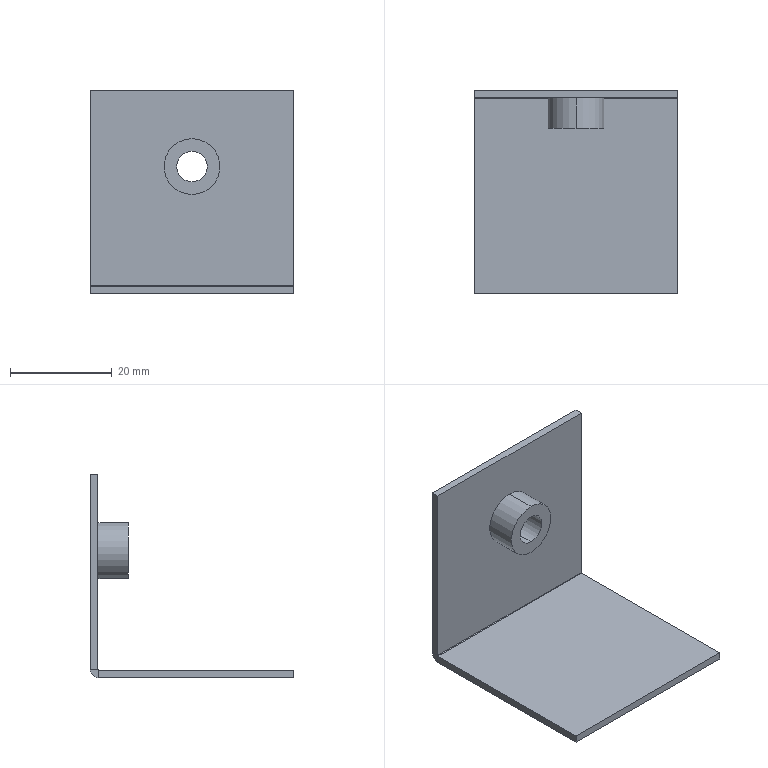Component | SolidWorks | CabinetWelding-1_MountingPlateBracket-1 | 1 solid | 22 faces | box 40 x 40 x 40 mm | volume 5013 mm3 | plane 14 | cylinder 8 | commonest cylinder face diameters 6 x2 11 x2 8 x2 3.2 x1 0.2 x1
STEP:
#1=CARTESIAN_POINT('',(11.302,-36.788,54.063));
#2=VERTEX_POINT('',#1);
#3=CARTESIAN_POINT('',(11.302,-36.788,54.299));
#4=VERTEX_POINT('',#3);
#5=CARTESIAN_POINT('',(11.302,-36.788,54.181));
#6=DIRECTION('',(0.,-1.,-0.));
#7=DIRECTION('',(0.,0.,1.));
#8=AXIS2_PLACEMENT_3D('',#5,#6,#7);
#9=CIRCLE('',#8,0.1181);
#10=EDGE_CURVE('',#2,#4,#9,.T.);
#11=ORIENTED_EDGE('',*,*,#10,.T.);
#12=CARTESIAN_POINT('',(11.302,-36.552,54.299));
#13=VERTEX_POINT('',#12);
#14=CARTESIAN_POINT('',(11.302,-36.788,54.299));
#15=DIRECTION('',(-0.,1.,0.));
#16=VECTOR('',#15,39.37);
#17=LINE('',#14,#16);
#18=EDGE_CURVE('',#4,#13,#17,.T.);
#19=ORIENTED_EDGE('',*,*,#18,.T.);
#20=CARTESIAN_POINT('',(11.302,-36.552,54.063));
#21=VERTEX_POINT('',#20);
#22=CARTESIAN_POINT('',(11.302,-36.552,54.181));
#23=DIRECTION('',(0.,-1.,-0.));
#24=DIRECTION('',(0.,0.,1.));
#25=AXIS2_PLACEMENT_3D('',#22,#23,#24);
#26=CIRCLE('',#25,0.1181);
#27=EDGE_CURVE('',#21,#13,#26,.T.);
#28=ORIENTED_EDGE('',*,*,#27,.F.);
#29=CARTESIAN_POINT('',(11.302,-36.788,54.063));
#30=DIRECTION('',(-0.,1.,0.));
#31=VECTOR('',#30,39.37);
#32=LINE('',#29,#31);
#33=EDGE_CURVE('',#2,#21,#32,.T.);
#34=ORIENTED_EDGE('',*,*,#33,.F.);
#35=EDGE_LOOP('',(#11,#19,#28,#34));
#36=FACE_OUTER_BOUND('',#35,.T.);
#37=CARTESIAN_POINT('',(11.302,-36.788,54.181));
#38=DIRECTION('',(-0.,1.,0.));
#39=DIRECTION('',(0.,0.,-1.));
#40=AXIS2_PLACEMENT_3D('',#37,#38,#39);
#41=CYLINDRICAL_SURFACE('',#40,0.1181);
#42=ADVANCED_FACE('',(#36),#41,.F.);
#43=CARTESIAN_POINT('',(11.302,-36.788,54.398));
#44=VERTEX_POINT('',#43);
#45=CARTESIAN_POINT('',(11.302,-36.788,53.965));
#46=VERTEX_POINT('',#45);
#47=CARTESIAN_POINT('',(11.302,-36.788,54.181));
#48=DIRECTION('',(0.,-1.,-0.));
#49=DIRECTION('',(0.,0.,1.));
#50=AXIS2_PLACEMENT_3D('',#47,#48,#49);
#51=CIRCLE('',#50,0.2165);
#52=EDGE_CURVE('',#44,#46,#51,.T.);
#53=ORIENTED_EDGE('',*,*,#52,.F.);
#54=CARTESIAN_POINT('',(11.302,-36.552,54.398));
#55=VERTEX_POINT('',#54);
#56=CARTESIAN_POINT('',(11.302,-36.788,54.398));
#57=DIRECTION('',(-0.,1.,0.));
#58=VECTOR('',#57,39.37);
#59=LINE('',#56,#58);
#60=EDGE_CURVE('',#44,#55,#59,.T.);
#61=ORIENTED_EDGE('',*,*,#60,.T.);
#62=CARTESIAN_POINT('',(11.302,-36.552,53.965));
#63=VERTEX_POINT('',#62);
#64=CARTESIAN_POINT('',(11.302,-36.552,54.181));
#65=DIRECTION('',(0.,-1.,-0.));
#66=DIRECTION('',(-1.,0.,0.));
#67=AXIS2_PLACEMENT_3D('',#64,#65,#66);
#68=CIRCLE('',#67,0.2165);
#69=EDGE_CURVE('',#55,#63,#68,.T.);
#70=ORIENTED_EDGE('',*,*,#69,.T.);
#71=CARTESIAN_POINT('',(11.302,-36.788,53.965));
#72=DIRECTION('',(-0.,1.,0.));
#73=VECTOR('',#72,39.37);
#74=LINE('',#71,#73);
#75=EDGE_CURVE('',#46,#63,#74,.T.);
#76=ORIENTED_EDGE('',*,*,#75,.F.);
#77=EDGE_LOOP('',(#53,#61,#70,#76));
#78=FACE_OUTER_BOUND('',#77,.T.);
#79=CARTESIAN_POINT('',(11.302,-36.788,54.181));
#80=DIRECTION('',(-0.,1.,0.));
#81=DIRECTION('',(-0.,0.,-1.));
#82=AXIS2_PLACEMENT_3D('',#79,#80,#81);
#83=CYLINDRICAL_SURFACE('',#82,0.2165);
#84=ADVANCED_FACE('',(#78),#83,.T.);
#85=CARTESIAN_POINT('',(11.46,-36.552,54.181));
#86=VERTEX_POINT('',#85);
#87=CARTESIAN_POINT('',(11.145,-36.552,54.181));
#88=VERTEX_POINT('',#87);
#89=CARTESIAN_POINT('',(11.302,-36.552,54.181));
#90=DIRECTION('',(-0.,1.,0.));
#91=DIRECTION('',(-1.,0.,0.));
#92=AXIS2_PLACEMENT_3D('',#89,#90,#91);
#93=CIRCLE('',#92,0.1575);
#94=EDGE_CURVE('',#86,#88,#93,.T.);
#95=ORIENTED_EDGE('',*,*,#94,.F.);
#96=CARTESIAN_POINT('',(11.46,-36.493,54.181));
#97=VERTEX_POINT('',#96);
#98=CARTESIAN_POINT('',(11.46,-36.887,54.181));
#99=DIRECTION('',(-0.,1.,0.));
#100=VECTOR('',#99,39.37);
#101=LINE('',#98,#100);
#102=EDGE_CURVE('',#86,#97,#101,.T.);
#103=ORIENTED_EDGE('',*,*,#102,.T.);
#104=CARTESIAN_POINT('',(11.145,-36.493,54.181));
#105=VERTEX_POINT('',#104);
#106=CARTESIAN_POINT('',(11.302,-36.493,54.181));
#107=DIRECTION('',(-0.,1.,0.));
#108=DIRECTION('',(-1.,0.,0.));
#109=AXIS2_PLACEMENT_3D('',#106,#107,#108);
#110=CIRCLE('',#109,0.1575);
#111=EDGE_CURVE('',#97,#105,#110,.T.);
#112=ORIENTED_EDGE('',*,*,#111,.T.);
#113=CARTESIAN_POINT('',(11.145,-36.887,54.181));
#114=DIRECTION('',(-0.,1.,0.));
#115=VECTOR('',#114,39.37);
#116=LINE('',#113,#115);
#117=EDGE_CURVE('',#88,#105,#116,.T.);
#118=ORIENTED_EDGE('',*,*,#117,.F.);
#119=EDGE_LOOP('',(#95,#103,#112,#118));
#120=FACE_OUTER_BOUND('',#119,.T.);
#121=CARTESIAN_POINT('',(11.302,-36.887,54.181));
#122=DIRECTION('',(-0.,1.,0.));
#123=DIRECTION('',(-1.,0.,0.));
#124=AXIS2_PLACEMENT_3D('',#121,#122,#123);
#125=CYLINDRICAL_SURFACE('',#124,0.1575);
#126=ADVANCED_FACE('',(#120),#125,.F.);
#127=CARTESIAN_POINT('',(12.09,-36.552,53.26));
#128=VERTEX_POINT('',#127);
#129=CARTESIAN_POINT('',(10.515,-36.552,53.26));
#130=VERTEX_POINT('',#129);
#131=CARTESIAN_POINT('',(12.09,-36.552,53.26));
#132=DIRECTION('',(-1.,-0.,0.));
#133=VECTOR('',#132,39.37);
#134=LINE('',#131,#133);
#135=EDGE_CURVE('',#128,#130,#134,.T.);
#136=ORIENTED_EDGE('',*,*,#135,.F.);
#137=CARTESIAN_POINT('',(12.09,-36.552,54.772));
#138=VERTEX_POINT('',#137);
#139=CARTESIAN_POINT('',(12.09,-36.552,54.772));
#140=DIRECTION('',(-0.,0.,-1.));
#141=VECTOR('',#140,39.37);
#142=LINE('',#139,#141);
#143=EDGE_CURVE('',#138,#128,#142,.T.);
#144=ORIENTED_EDGE('',*,*,#143,.F.);
#145=CARTESIAN_POINT('',(10.515,-36.552,54.772));
#146=VERTEX_POINT('',#145);
#147=CARTESIAN_POINT('',(12.09,-36.552,54.772));
#148=DIRECTION('',(1.,0.,-0.));
#149=VECTOR('',#148,39.37);
#150=LINE('',#147,#149);
#151=EDGE_CURVE('',#146,#138,#150,.T.);
#152=ORIENTED_EDGE('',*,*,#151,.F.);
#153=CARTESIAN_POINT('',(10.515,-36.552,54.772));
#154=DIRECTION('',(0.,-0.,1.));
#155=VECTOR('',#154,39.37);
#156=LINE('',#153,#155);
#157=EDGE_CURVE('',#130,#146,#156,.T.);
#158=ORIENTED_EDGE('',*,*,#157,.F.);
#159=EDGE_LOOP('',(#136,#144,#152,#158));
#160=FACE_OUTER_BOUND('',#159,.T.);
#161=CARTESIAN_POINT('',(11.302,-36.552,54.181));
#162=DIRECTION('',(0.,-1.,-0.));
#163=DIRECTION('',(-1.,0.,0.));
#164=AXIS2_PLACEMENT_3D('',#161,#162,#163);
#165=CIRCLE('',#164,0.2165);
#166=EDGE_CURVE('',#63,#55,#165,.T.);
#167=ORIENTED_EDGE('',*,*,#166,.F.);
#168=ORIENTED_EDGE('',*,*,#69,.F.);
#169=EDGE_LOOP('',(#167,#168));
#170=FACE_BOUND('',#169,.T.);
#171=CARTESIAN_POINT('',(11.33,-36.552,53.333));
#172=DIRECTION('',(-0.,1.,0.));
#173=DIRECTION('',(-1.,-0.,0.));
#174=AXIS2_PLACEMENT_3D('',#171,#172,#173);
#175=PLANE('',#174);
#176=ADVANCED_FACE('',(#160,#170),#175,.F.);
#177=ORIENTED_EDGE('',*,*,#143,.T.);
#178=CARTESIAN_POINT('',(12.09,-36.493,53.26));
#179=VERTEX_POINT('',#178);
#180=CARTESIAN_POINT('',(12.09,-36.552,53.26));
#181=DIRECTION('',(-0.,1.,0.));
#182=VECTOR('',#181,39.37);
#183=LINE('',#180,#182);
#184=EDGE_CURVE('',#128,#179,#183,.T.);
#185=ORIENTED_EDGE('',*,*,#184,.T.);
#186=CARTESIAN_POINT('',(12.09,-36.493,54.772));
#187=VERTEX_POINT('',#186);
#188=CARTESIAN_POINT('',(12.09,-36.493,54.772));
#189=DIRECTION('',(-0.,0.,-1.));
#190=VECTOR('',#189,39.37);
#191=LINE('',#188,#190);
#192=EDGE_CURVE('',#187,#179,#191,.T.);
#193=ORIENTED_EDGE('',*,*,#192,.F.);
#194=CARTESIAN_POINT('',(12.09,-36.552,54.772));
#195=DIRECTION('',(-0.,1.,0.));
#196=VECTOR('',#195,39.37);
#197=LINE('',#194,#196);
#198=EDGE_CURVE('',#138,#187,#197,.T.);
#199=ORIENTED_EDGE('',*,*,#198,.F.);
#200=EDGE_LOOP('',(#177,#185,#193,#199));
#201=FACE_OUTER_BOUND('',#200,.T.);
#202=CARTESIAN_POINT('',(12.09,-36.552,54.772));
#203=DIRECTION('',(1.,0.,-0.));
#204=DIRECTION('',(-0.,0.,-1.));
#205=AXIS2_PLACEMENT_3D('',#202,#203,#204);
#206=PLANE('',#205);
#207=ADVANCED_FACE('',(#201),#206,.T.);
#208=CARTESIAN_POINT('',(11.302,-36.493,54.181));
#209=DIRECTION('',(-0.,1.,0.));
#210=DIRECTION('',(-1.,0.,0.));
#211=AXIS2_PLACEMENT_3D('',#208,#209,#210);
#212=CIRCLE('',#211,0.1575);
#213=EDGE_CURVE('',#105,#97,#212,.T.);
#214=ORIENTED_EDGE('',*,*,#213,.F.);
#215=ORIENTED_EDGE('',*,*,#111,.F.);
#216=EDGE_LOOP('',(#214,#215));
#217=FACE_BOUND('',#216,.T.);
#218=ORIENTED_EDGE('',*,*,#192,.T.);
#219=CARTESIAN_POINT('',(10.515,-36.493,53.26));
#220=VERTEX_POINT('',#219);
#221=CARTESIAN_POINT('',(12.09,-36.493,53.26));
#222=DIRECTION('',(-1.,-0.,0.));
#223=VECTOR('',#222,39.37);
#224=LINE('',#221,#223);
#225=EDGE_CURVE('',#179,#220,#224,.T.);
#226=ORIENTED_EDGE('',*,*,#225,.T.);
#227=CARTESIAN_POINT('',(10.515,-36.493,54.772));
#228=VERTEX_POINT('',#227);
#229=CARTESIAN_POINT('',(10.515,-36.493,54.772));
#230=DIRECTION('',(0.,-0.,1.));
#231=VECTOR('',#230,39.37);
#232=LINE('',#229,#231);
#233=EDGE_CURVE('',#220,#228,#232,.T.);
#234=ORIENTED_EDGE('',*,*,#233,.T.);
#235=CARTESIAN_POINT('',(12.09,-36.493,54.772));
#236=DIRECTION('',(1.,0.,-0.));
#237=VECTOR('',#236,39.37);
#238=LINE('',#235,#237);
#239=EDGE_CURVE('',#228,#187,#238,.T.);
#240=ORIENTED_EDGE('',*,*,#239,.T.);
#241=EDGE_LOOP('',(#218,#226,#234,#240));
#242=FACE_OUTER_BOUND('',#241,.T.);
#243=CARTESIAN_POINT('',(11.33,-36.493,53.333));
#244=DIRECTION('',(-0.,1.,0.));
#245=DIRECTION('',(-1.,-0.,0.));
#246=AXIS2_PLACEMENT_3D('',#243,#244,#245);
#247=PLANE('',#246);
#248=ADVANCED_FACE('',(#217,#242),#247,.T.);
#249=ORIENTED_EDGE('',*,*,#239,.F.);
#250=CARTESIAN_POINT('',(10.515,-36.552,54.772));
#251=DIRECTION('',(-0.,1.,0.));
#252=VECTOR('',#251,39.37);
#253=LINE('',#250,#252);
#254=EDGE_CURVE('',#146,#228,#253,.T.);
#255=ORIENTED_EDGE('',*,*,#254,.F.);
#256=ORIENTED_EDGE('',*,*,#151,.T.);
#257=ORIENTED_EDGE('',*,*,#198,.T.);
#258=EDGE_LOOP('',(#249,#255,#256,#257));
#259=FACE_OUTER_BOUND('',#258,.T.);
#260=CARTESIAN_POINT('',(12.09,-36.552,54.772));
#261=DIRECTION('',(0.,-0.,1.));
#262=DIRECTION('',(-0.,1.,0.));
#263=AXIS2_PLACEMENT_3D('',#260,#261,#262);
#264=PLANE('',#263);
#265=ADVANCED_FACE('',(#259),#264,.T.);
#266=CARTESIAN_POINT('',(10.515,-36.552,53.26));
#267=DIRECTION('',(-0.,1.,0.));
#268=VECTOR('',#267,39.37);
#269=LINE('',#266,#268);
#270=EDGE_CURVE('',#130,#220,#269,.T.);
#271=ORIENTED_EDGE('',*,*,#270,.F.);
#272=ORIENTED_EDGE('',*,*,#157,.T.);
#273=ORIENTED_EDGE('',*,*,#254,.T.);
#274=ORIENTED_EDGE('',*,*,#233,.F.);
#275=EDGE_LOOP('',(#271,#272,#273,#274));
#276=FACE_OUTER_BOUND('',#275,.T.);
#277=CARTESIAN_POINT('',(10.515,-36.552,54.772));
#278=DIRECTION('',(-1.,-0.,0.));
#279=DIRECTION('',(0.,-0.,1.));
#280=AXIS2_PLACEMENT_3D('',#277,#278,#279);
#281=PLANE('',#280);
#282=ADVANCED_FACE('',(#276),#281,.T.);
#283=CARTESIAN_POINT('',(10.515,-36.556,53.256));
#284=VERTEX_POINT('',#283);
#285=CARTESIAN_POINT('',(10.515,-36.556,53.197));
#286=VERTEX_POINT('',#285);
#287=CARTESIAN_POINT('',(10.515,-36.556,53.197));
#288=DIRECTION('',(-0.,0.,-1.));
#289=VECTOR('',#288,39.37);
#290=LINE('',#287,#289);
#291=EDGE_CURVE('',#284,#286,#290,.T.);
#292=ORIENTED_EDGE('',*,*,#291,.F.);
#293=CARTESIAN_POINT('',(10.515,-36.556,53.26));
#294=DIRECTION('',(-1.,-0.,0.));
#295=DIRECTION('',(0.,1.,0.));
#296=AXIS2_PLACEMENT_3D('',#293,#294,#295);
#297=CIRCLE('',#296,0.003937);
#298=EDGE_CURVE('',#130,#284,#297,.T.);
#299=ORIENTED_EDGE('',*,*,#298,.F.);
#300=ORIENTED_EDGE('',*,*,#270,.T.);
#301=CARTESIAN_POINT('',(10.515,-36.556,53.26));
#302=DIRECTION('',(-1.,-0.,0.));
#303=DIRECTION('',(0.,1.,0.));
#304=AXIS2_PLACEMENT_3D('',#301,#302,#303);
#305=CIRCLE('',#304,0.06299);
#306=EDGE_CURVE('',#220,#286,#305,.T.);
#307=ORIENTED_EDGE('',*,*,#306,.T.);
#308=EDGE_LOOP('',(#292,#299,#300,#307));
#309=FACE_OUTER_BOUND('',#308,.T.);
#310=CARTESIAN_POINT('',(10.515,-36.556,53.26));
#311=DIRECTION('',(-1.,-0.,0.));
#312=DIRECTION('',(0.,-1.,-0.));
#313=AXIS2_PLACEMENT_3D('',#310,#311,#312);
#314=PLANE('',#313);
#315=ADVANCED_FACE('',(#309),#314,.T.);
#316=CARTESIAN_POINT('',(12.09,-36.556,53.256));
#317=VERTEX_POINT('',#316);
#318=CARTESIAN_POINT('',(12.09,-36.556,53.26));
#319=DIRECTION('',(1.,0.,-0.));
#320=DIRECTION('',(0.,1.,0.));
#321=AXIS2_PLACEMENT_3D('',#318,#319,#320);
#322=CIRCLE('',#321,0.003937);
#323=EDGE_CURVE('',#317,#128,#322,.T.);
#324=ORIENTED_EDGE('',*,*,#323,.F.);
#325=CARTESIAN_POINT('',(12.09,-36.556,53.197));
#326=VERTEX_POINT('',#325);
#327=CARTESIAN_POINT('',(12.09,-36.556,53.256));
#328=DIRECTION('',(-0.,0.,-1.));
#329=VECTOR('',#328,39.37);
#330=LINE('',#327,#329);
#331=EDGE_CURVE('',#317,#326,#330,.T.);
#332=ORIENTED_EDGE('',*,*,#331,.T.);
#333=CARTESIAN_POINT('',(12.09,-36.556,53.26));
#334=DIRECTION('',(1.,0.,-0.));
#335=DIRECTION('',(0.,1.,0.));
#336=AXIS2_PLACEMENT_3D('',#333,#334,#335);
#337=CIRCLE('',#336,0.06299);
#338=EDGE_CURVE('',#326,#179,#337,.T.);
#339=ORIENTED_EDGE('',*,*,#338,.T.);
#340=ORIENTED_EDGE('',*,*,#184,.F.);
#341=EDGE_LOOP('',(#324,#332,#339,#340));
#342=FACE_OUTER_BOUND('',#341,.T.);
#343=CARTESIAN_POINT('',(12.09,-36.556,53.26));
#344=DIRECTION('',(-1.,-0.,0.));
#345=DIRECTION('',(0.,-1.,-0.));
#346=AXIS2_PLACEMENT_3D('',#343,#344,#345);
#347=PLANE('',#346);
#348=ADVANCED_FACE('',(#342),#347,.F.);
#349=ORIENTED_EDGE('',*,*,#225,.F.);
#350=ORIENTED_EDGE('',*,*,#338,.F.);
#351=CARTESIAN_POINT('',(11.33,-36.556,53.197));
#352=DIRECTION('',(1.,0.,-0.));
#353=VECTOR('',#352,39.37);
#354=LINE('',#351,#353);
#355=EDGE_CURVE('',#286,#326,#354,.T.);
#356=ORIENTED_EDGE('',*,*,#355,.F.);
#357=ORIENTED_EDGE('',*,*,#306,.F.);
#358=EDGE_LOOP('',(#349,#350,#356,#357));
#359=FACE_OUTER_BOUND('',#358,.T.);
#360=CARTESIAN_POINT('',(12.09,-36.556,53.26));
#361=DIRECTION('',(1.,0.,-0.));
#362=DIRECTION('',(0.,0.,-1.));
#363=AXIS2_PLACEMENT_3D('',#360,#361,#362);
#364=CYLINDRICAL_SURFACE('',#363,0.06299);
#365=ADVANCED_FACE('',(#359),#364,.T.);
#366=ORIENTED_EDGE('',*,*,#135,.T.);
#367=ORIENTED_EDGE('',*,*,#298,.T.);
#368=CARTESIAN_POINT('',(10.515,-36.556,53.256));
#369=DIRECTION('',(1.,0.,-0.));
#370=VECTOR('',#369,39.37);
#371=LINE('',#368,#370);
#372=EDGE_CURVE('',#284,#317,#371,.T.);
#373=ORIENTED_EDGE('',*,*,#372,.T.);
#374=ORIENTED_EDGE('',*,*,#323,.T.);
#375=EDGE_LOOP('',(#366,#367,#373,#374));
#376=FACE_OUTER_BOUND('',#375,.T.);
#377=CARTESIAN_POINT('',(12.09,-36.556,53.26));
#378=DIRECTION('',(1.,0.,-0.));
#379=DIRECTION('',(0.,0.,-1.));
#380=AXIS2_PLACEMENT_3D('',#377,#378,#379);
#381=CYLINDRICAL_SURFACE('',#380,0.003937);
#382=ADVANCED_FACE('',(#376),#381,.F.);
#383=CARTESIAN_POINT('',(12.09,-38.068,53.197));
#384=VERTEX_POINT('',#383);
#385=CARTESIAN_POINT('',(12.09,-36.552,53.197));
#386=DIRECTION('',(-0.,1.,0.));
#387=VECTOR('',#386,39.37);
#388=LINE('',#385,#387);
#389=EDGE_CURVE('',#384,#326,#388,.T.);
#390=ORIENTED_EDGE('',*,*,#389,.T.);
#391=ORIENTED_EDGE('',*,*,#331,.F.);
#392=CARTESIAN_POINT('',(12.09,-38.068,53.256));
#393=VERTEX_POINT('',#392);
#394=CARTESIAN_POINT('',(12.09,-36.493,53.256));
#395=DIRECTION('',(-0.,1.,0.));
#396=VECTOR('',#395,39.37);
#397=LINE('',#394,#396);
#398=EDGE_CURVE('',#393,#317,#397,.T.);
#399=ORIENTED_EDGE('',*,*,#398,.F.);
#400=CARTESIAN_POINT('',(12.09,-38.068,53.197));
#401=DIRECTION('',(0.,-0.,1.));
#402=VECTOR('',#401,39.37);
#403=LINE('',#400,#402);
#404=EDGE_CURVE('',#384,#393,#403,.T.);
#405=ORIENTED_EDGE('',*,*,#404,.F.);
#406=EDGE_LOOP('',(#390,#391,#399,#405));
#407=FACE_OUTER_BOUND('',#406,.T.);
#408=CARTESIAN_POINT('',(12.09,-36.552,53.197));
#409=DIRECTION('',(1.,0.,-0.));
#410=DIRECTION('',(-0.,1.,0.));
#411=AXIS2_PLACEMENT_3D('',#408,#409,#410);
#412=PLANE('',#411);
#413=ADVANCED_FACE('',(#407),#412,.T.);
#414=CARTESIAN_POINT('',(10.515,-38.068,53.256));
#415=VERTEX_POINT('',#414);
#416=CARTESIAN_POINT('',(10.515,-36.493,53.256));
#417=DIRECTION('',(0.,-1.,-0.));
#418=VECTOR('',#417,39.37);
#419=LINE('',#416,#418);
#420=EDGE_CURVE('',#284,#415,#419,.T.);
#421=ORIENTED_EDGE('',*,*,#420,.F.);
#422=ORIENTED_EDGE('',*,*,#291,.T.);
#423=CARTESIAN_POINT('',(10.515,-38.068,53.197));
#424=VERTEX_POINT('',#423);
#425=CARTESIAN_POINT('',(10.515,-38.068,53.197));
#426=DIRECTION('',(0.,-1.,-0.));
#427=VECTOR('',#426,39.37);
#428=LINE('',#425,#427);
#429=EDGE_CURVE('',#286,#424,#428,.T.);
#430=ORIENTED_EDGE('',*,*,#429,.T.);
#431=CARTESIAN_POINT('',(10.515,-38.068,53.197));
#432=DIRECTION('',(0.,-0.,1.));
#433=VECTOR('',#432,39.37);
#434=LINE('',#431,#433);
#435=EDGE_CURVE('',#424,#415,#434,.T.);
#436=ORIENTED_EDGE('',*,*,#435,.T.);
#437=EDGE_LOOP('',(#421,#422,#430,#436));
#438=FACE_OUTER_BOUND('',#437,.T.);
#439=CARTESIAN_POINT('',(10.515,-38.068,53.197));
#440=DIRECTION('',(-1.,-0.,0.));
#441=DIRECTION('',(0.,-1.,-0.));
#442=AXIS2_PLACEMENT_3D('',#439,#440,#441);
#443=PLANE('',#442);
#444=ADVANCED_FACE('',(#438),#443,.T.);
#445=ORIENTED_EDGE('',*,*,#429,.F.);
#446=ORIENTED_EDGE('',*,*,#355,.T.);
#447=ORIENTED_EDGE('',*,*,#389,.F.);
#448=CARTESIAN_POINT('',(12.09,-38.068,53.197));
#449=DIRECTION('',(1.,0.,-0.));
#450=VECTOR('',#449,39.37);
#451=LINE('',#448,#450);
#452=EDGE_CURVE('',#424,#384,#451,.T.);
#453=ORIENTED_EDGE('',*,*,#452,.F.);
#454=EDGE_LOOP('',(#445,#446,#447,#453));
#455=FACE_OUTER_BOUND('',#454,.T.);
#456=CARTESIAN_POINT('',(11.33,-36.493,53.197));
#457=DIRECTION('',(-0.,0.,-1.));
#458=DIRECTION('',(0.,-1.,-0.));
#459=AXIS2_PLACEMENT_3D('',#456,#457,#458);
#460=PLANE('',#459);
#461=ADVANCED_FACE('',(#455),#460,.T.);
#462=ORIENTED_EDGE('',*,*,#372,.F.);
#463=ORIENTED_EDGE('',*,*,#420,.T.);
#464=CARTESIAN_POINT('',(11.33,-38.068,53.256));
#465=DIRECTION('',(1.,0.,-0.));
#466=VECTOR('',#465,39.37);
#467=LINE('',#464,#466);
#468=EDGE_CURVE('',#415,#393,#467,.T.);
#469=ORIENTED_EDGE('',*,*,#468,.T.);
#470=ORIENTED_EDGE('',*,*,#398,.T.);
#471=EDGE_LOOP('',(#462,#463,#469,#470));
#472=FACE_OUTER_BOUND('',#471,.T.);
#473=CARTESIAN_POINT('',(11.33,-36.493,53.256));
#474=DIRECTION('',(-0.,0.,-1.));
#475=DIRECTION('',(0.,-1.,-0.));
#476=AXIS2_PLACEMENT_3D('',#473,#474,#475);
#477=PLANE('',#476);
#478=ADVANCED_FACE('',(#472),#477,.F.);
#479=ORIENTED_EDGE('',*,*,#468,.F.);
#480=ORIENTED_EDGE('',*,*,#435,.F.);
#481=ORIENTED_EDGE('',*,*,#452,.T.);
#482=ORIENTED_EDGE('',*,*,#404,.T.);
#483=EDGE_LOOP('',(#479,#480,#481,#482));
#484=FACE_OUTER_BOUND('',#483,.T.);
#485=CARTESIAN_POINT('',(12.09,-38.068,53.197));
#486=DIRECTION('',(0.,-1.,-0.));
#487=DIRECTION('',(0.,-0.,1.));
#488=AXIS2_PLACEMENT_3D('',#485,#486,#487);
#489=PLANE('',#488);
#490=ADVANCED_FACE('',(#484),#489,.T.);
#491=ORIENTED_EDGE('',*,*,#102,.F.);
#492=CARTESIAN_POINT('',(11.302,-36.552,54.181));
#493=DIRECTION('',(-0.,1.,0.));
#494=DIRECTION('',(-1.,0.,0.));
#495=AXIS2_PLACEMENT_3D('',#492,#493,#494);
#496=CIRCLE('',#495,0.1575);
#497=EDGE_CURVE('',#88,#86,#496,.T.);
#498=ORIENTED_EDGE('',*,*,#497,.F.);
#499=ORIENTED_EDGE('',*,*,#117,.T.);
#500=ORIENTED_EDGE('',*,*,#213,.T.);
#501=EDGE_LOOP('',(#491,#498,#499,#500));
#502=FACE_OUTER_BOUND('',#501,.T.);
#503=CARTESIAN_POINT('',(11.302,-36.887,54.181));
#504=DIRECTION('',(-0.,1.,0.));
#505=DIRECTION('',(-1.,0.,0.));
#506=AXIS2_PLACEMENT_3D('',#503,#504,#505);
#507=CYLINDRICAL_SURFACE('',#506,0.1575);
#508=ADVANCED_FACE('',(#502),#507,.F.);
#509=ORIENTED_EDGE('',*,*,#27,.T.);
#510=CARTESIAN_POINT('',(11.302,-36.552,54.181));
#511=DIRECTION('',(0.,-1.,-0.));
#512=DIRECTION('',(0.,0.,1.));
#513=AXIS2_PLACEMENT_3D('',#510,#511,#512);
#514=CIRCLE('',#513,0.1181);
#515=EDGE_CURVE('',#13,#21,#514,.T.);
#516=ORIENTED_EDGE('',*,*,#515,.T.);
#517=EDGE_LOOP('',(#509,#516));
#518=FACE_BOUND('',#517,.T.);
#519=ORIENTED_EDGE('',*,*,#497,.T.);
#520=ORIENTED_EDGE('',*,*,#94,.T.);
#521=EDGE_LOOP('',(#519,#520));
#522=FACE_OUTER_BOUND('',#521,.T.);
#523=CARTESIAN_POINT('',(11.302,-36.552,54.181));
#524=DIRECTION('',(0.,-1.,-0.));
#525=DIRECTION('',(0.,-0.,1.));
#526=AXIS2_PLACEMENT_3D('',#523,#524,#525);
#527=PLANE('',#526);
#528=ADVANCED_FACE('',(#518,#522),#527,.F.);
#529=CARTESIAN_POINT('',(11.302,-36.788,54.181));
#530=DIRECTION('',(0.,-1.,-0.));
#531=DIRECTION('',(0.,0.,1.));
#532=AXIS2_PLACEMENT_3D('',#529,#530,#531);
#533=CIRCLE('',#532,0.2165);
#534=EDGE_CURVE('',#46,#44,#533,.T.);
#535=ORIENTED_EDGE('',*,*,#534,.T.);
#536=ORIENTED_EDGE('',*,*,#52,.T.);
#537=EDGE_LOOP('',(#535,#536));
#538=FACE_OUTER_BOUND('',#537,.T.);
#539=ORIENTED_EDGE('',*,*,#10,.F.);
#540=CARTESIAN_POINT('',(11.302,-36.788,54.181));
#541=DIRECTION('',(0.,-1.,-0.));
#542=DIRECTION('',(0.,0.,1.));
#543=AXIS2_PLACEMENT_3D('',#540,#541,#542);
#544=CIRCLE('',#543,0.1181);
#545=EDGE_CURVE('',#4,#2,#544,.T.);
#546=ORIENTED_EDGE('',*,*,#545,.F.);
#547=EDGE_LOOP('',(#539,#546));
#548=FACE_BOUND('',#547,.T.);
#549=CARTESIAN_POINT('',(11.302,-36.788,54.181));
#550=DIRECTION('',(0.,-1.,-0.));
#551=DIRECTION('',(0.,-0.,1.));
#552=AXIS2_PLACEMENT_3D('',#549,#550,#551);
#553=PLANE('',#552);
#554=ADVANCED_FACE('',(#538,#548),#553,.T.);
#555=ORIENTED_EDGE('',*,*,#60,.F.);
#556=ORIENTED_EDGE('',*,*,#534,.F.);
#557=ORIENTED_EDGE('',*,*,#75,.T.);
#558=ORIENTED_EDGE('',*,*,#166,.T.);
#559=EDGE_LOOP('',(#555,#556,#557,#558));
#560=FACE_OUTER_BOUND('',#559,.T.);
#561=CARTESIAN_POINT('',(11.302,-36.788,54.181));
#562=DIRECTION('',(-0.,1.,0.));
#563=DIRECTION('',(-0.,0.,-1.));
#564=AXIS2_PLACEMENT_3D('',#561,#562,#563);
#565=CYLINDRICAL_SURFACE('',#564,0.2165);
#566=ADVANCED_FACE('',(#560),#565,.T.);
#567=ORIENTED_EDGE('',*,*,#18,.F.);
#568=ORIENTED_EDGE('',*,*,#545,.T.);
#569=ORIENTED_EDGE('',*,*,#33,.T.);
#570=ORIENTED_EDGE('',*,*,#515,.F.);
#571=EDGE_LOOP('',(#567,#568,#569,#570));
#572=FACE_OUTER_BOUND('',#571,.T.);
#573=CARTESIAN_POINT('',(11.302,-36.788,54.181));
#574=DIRECTION('',(-0.,1.,0.));
#575=DIRECTION('',(0.,0.,-1.));
#576=AXIS2_PLACEMENT_3D('',#573,#574,#575);
#577=CYLINDRICAL_SURFACE('',#576,0.1181);
#578=ADVANCED_FACE('',(#572),#577,.F.);
#579=CLOSED_SHELL('',(#42,#84,#126,#176,#207,#248,#265,#282,#315,#348,#365,#382,#413,#444,#461,#478,#490,#508,#528,#554,#566,#578));
#580=MANIFOLD_SOLID_BREP('',#579);
#581=CARTESIAN_POINT('',(0.,0.,0.));
#582=DIRECTION('',(0.,0.,1.));
#583=DIRECTION('',(1.,0.,0.));
#584=AXIS2_PLACEMENT_3D('',#581,#582,#583);
#585=(LENGTH_UNIT()NAMED_UNIT(*)SI_UNIT($,.METRE.));
#586=LENGTH_MEASURE_WITH_UNIT(LENGTH_MEASURE(0.0254),#585);
#587=DIMENSIONAL_EXPONENTS(1.,0.,0.,0.,0.,0.,0.);
#588=(CONVERSION_BASED_UNIT('',#586)LENGTH_UNIT()NAMED_UNIT(#587));
#589=UNCERTAINTY_MEASURE_WITH_UNIT(LENGTH_MEASURE(0.00001),#588,'','');
#590=(NAMED_UNIT(*)PLANE_ANGLE_UNIT()SI_UNIT($,.RADIAN.));
#591=(NAMED_UNIT(*)SI_UNIT($,.STERADIAN.)SOLID_ANGLE_UNIT());
#592=(GEOMETRIC_REPRESENTATION_CONTEXT(3)GLOBAL_UNCERTAINTY_ASSIGNED_CONTEXT((#589))GLOBAL_UNIT_ASSIGNED_CONTEXT((#588,#590,#591))REPRESENTATION_CONTEXT('',''));
#593=ADVANCED_BREP_SHAPE_REPRESENTATION('',(#580,#584),#592);
#594=COLOUR_RGB('',0.7922,0.8196,0.9333);
#595=FILL_AREA_STYLE_COLOUR('',#594);
#596=FILL_AREA_STYLE('',(#595));
#597=SURFACE_STYLE_FILL_AREA(#596);
#598=SURFACE_SIDE_STYLE('',(#597));
#599=SURFACE_STYLE_USAGE(.BOTH.,#598);
#600=PRESENTATION_STYLE_ASSIGNMENT((#599));
#601=STYLED_ITEM('',(#600),#580);
#602=PRESENTATION_LAYER_ASSIGNMENT('','',(#601));
#603=(LENGTH_UNIT()NAMED_UNIT(*)SI_UNIT($,.METRE.));
#604=LENGTH_MEASURE_WITH_UNIT(LENGTH_MEASURE(0.0254),#603);
#605=DIMENSIONAL_EXPONENTS(1.,0.,0.,0.,0.,0.,0.);
#606=(CONVERSION_BASED_UNIT('',#604)LENGTH_UNIT()NAMED_UNIT(#605));
#607=UNCERTAINTY_MEASURE_WITH_UNIT(LENGTH_MEASURE(0.00001),#606,'','');
#608=(NAMED_UNIT(*)PLANE_ANGLE_UNIT()SI_UNIT($,.RADIAN.));
#609=(NAMED_UNIT(*)SI_UNIT($,.STERADIAN.)SOLID_ANGLE_UNIT());
#610=(GEOMETRIC_REPRESENTATION_CONTEXT(3)GLOBAL_UNCERTAINTY_ASSIGNED_CONTEXT((#607))GLOBAL_UNIT_ASSIGNED_CONTEXT((#606,#608,#609))REPRESENTATION_CONTEXT('',''));
#611=MECHANICAL_DESIGN_GEOMETRIC_PRESENTATION_REPRESENTATION('',(#601),#610);